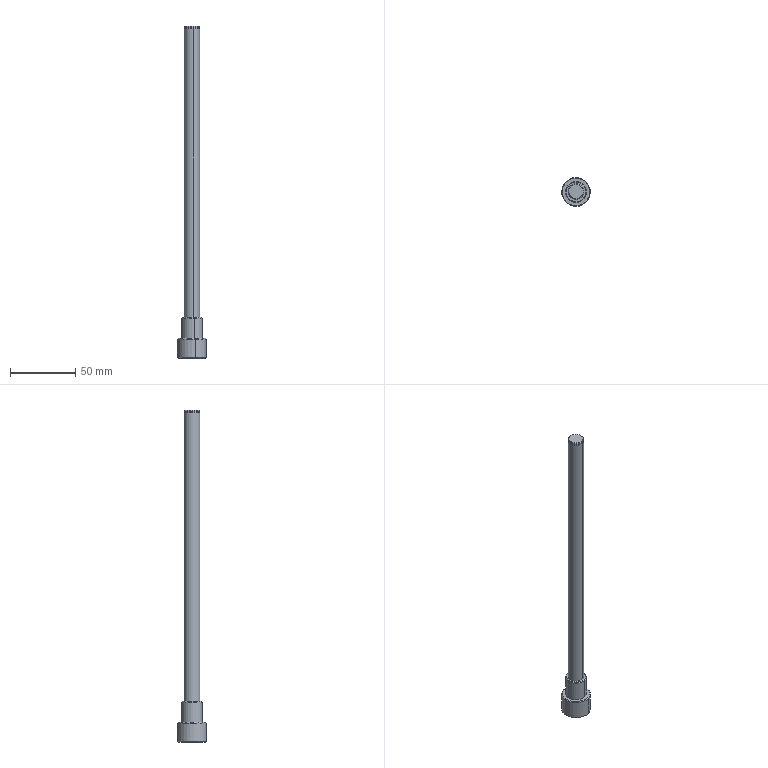Component | SolidWorks | JYTBJ-HeaderRollerBody-1_JYTBJ-HeaderRollerAxis-1 | 1 solid | 28 faces | box 22 x 22 x 254 mm | volume 33731 mm3 | cylinder 12 | cone 10 | plane 6 | commonest cylinder face diameters 12 x4 11 x2 5 x2 16 x2 22 x2
STEP:
#1=COLOUR_RGB('',0.7922,0.8196,0.9333);
#2=FILL_AREA_STYLE_COLOUR('',#1);
#3=FILL_AREA_STYLE('',(#2));
#4=SURFACE_STYLE_FILL_AREA(#3);
#5=SURFACE_SIDE_STYLE('',(#4));
#6=SURFACE_STYLE_USAGE(.BOTH.,#5);
#7=PRESENTATION_STYLE_ASSIGNMENT((#6));
#8=CARTESIAN_POINT('',(-7.808,6.896,10.63));
#9=VERTEX_POINT('',#8);
#10=CARTESIAN_POINT('',(-7.915,7.357,10.63));
#11=VERTEX_POINT('',#10);
#12=CARTESIAN_POINT('',(-7.862,7.126,10.63));
#13=DIRECTION('',(-0.,0.,-1.));
#14=DIRECTION('',(0.2266,-0.974,0.));
#15=AXIS2_PLACEMENT_3D('',#12,#13,#14);
#16=CIRCLE('',#15,0.2362);
#17=EDGE_CURVE('',#9,#11,#16,.T.);
#18=ORIENTED_EDGE('',*,*,#17,.T.);
#19=CARTESIAN_POINT('',(-7.915,7.357,1.929));
#20=VERTEX_POINT('',#19);
#21=CARTESIAN_POINT('',(-7.915,7.357,10.394));
#22=DIRECTION('',(-0.,0.,-1.));
#23=VECTOR('',#22,39.37);
#24=LINE('',#21,#23);
#25=EDGE_CURVE('',#11,#20,#24,.T.);
#26=ORIENTED_EDGE('',*,*,#25,.T.);
#27=CARTESIAN_POINT('',(-7.808,6.896,1.929));
#28=VERTEX_POINT('',#27);
#29=CARTESIAN_POINT('',(-7.862,7.126,1.929));
#30=DIRECTION('',(0.,-0.,1.));
#31=DIRECTION('',(-0.2266,0.974,0.));
#32=AXIS2_PLACEMENT_3D('',#29,#30,#31);
#33=CIRCLE('',#32,0.2362);
#34=EDGE_CURVE('',#20,#28,#33,.T.);
#35=ORIENTED_EDGE('',*,*,#34,.T.);
#36=CARTESIAN_POINT('',(-7.808,6.896,10.394));
#37=DIRECTION('',(-0.,0.,-1.));
#38=VECTOR('',#37,39.37);
#39=LINE('',#36,#38);
#40=EDGE_CURVE('',#9,#28,#39,.T.);
#41=ORIENTED_EDGE('',*,*,#40,.F.);
#42=EDGE_LOOP('',(#18,#26,#35,#41));
#43=FACE_OUTER_BOUND('',#42,.T.);
#44=CARTESIAN_POINT('',(-7.862,7.126,10.394));
#45=DIRECTION('',(-0.,0.,-1.));
#46=DIRECTION('',(0.2266,-0.974,0.));
#47=AXIS2_PLACEMENT_3D('',#44,#45,#46);
#48=CYLINDRICAL_SURFACE('',#47,0.2362);
#49=ADVANCED_FACE('',(#43),#48,.T.);
#50=CARTESIAN_POINT('',(-7.911,7.337,10.63));
#51=VERTEX_POINT('',#50);
#52=CARTESIAN_POINT('',(-7.813,6.916,10.63));
#53=VERTEX_POINT('',#52);
#54=CARTESIAN_POINT('',(-7.862,7.126,10.63));
#55=DIRECTION('',(0.,-0.,1.));
#56=DIRECTION('',(-0.2266,0.974,0.));
#57=AXIS2_PLACEMENT_3D('',#54,#55,#56);
#58=CIRCLE('',#57,0.2165);
#59=EDGE_CURVE('',#51,#53,#58,.T.);
#60=ORIENTED_EDGE('',*,*,#59,.T.);
#61=CARTESIAN_POINT('',(-7.813,6.916,10.669));
#62=VERTEX_POINT('',#61);
#63=CARTESIAN_POINT('',(-7.813,6.916,10.709));
#64=DIRECTION('',(0.,-0.,1.));
#65=VECTOR('',#64,39.37);
#66=LINE('',#63,#65);
#67=EDGE_CURVE('',#53,#62,#66,.T.);
#68=ORIENTED_EDGE('',*,*,#67,.T.);
#69=CARTESIAN_POINT('',(-7.911,7.337,10.669));
#70=VERTEX_POINT('',#69);
#71=CARTESIAN_POINT('',(-7.862,7.126,10.669));
#72=DIRECTION('',(0.,-0.,1.));
#73=DIRECTION('',(-0.2266,0.974,0.));
#74=AXIS2_PLACEMENT_3D('',#71,#72,#73);
#75=CIRCLE('',#74,0.2165);
#76=EDGE_CURVE('',#70,#62,#75,.T.);
#77=ORIENTED_EDGE('',*,*,#76,.F.);
#78=CARTESIAN_POINT('',(-7.911,7.337,10.709));
#79=DIRECTION('',(0.,-0.,1.));
#80=VECTOR('',#79,39.37);
#81=LINE('',#78,#80);
#82=EDGE_CURVE('',#51,#70,#81,.T.);
#83=ORIENTED_EDGE('',*,*,#82,.F.);
#84=EDGE_LOOP('',(#60,#68,#77,#83));
#85=FACE_OUTER_BOUND('',#84,.T.);
#86=CARTESIAN_POINT('',(-7.862,7.126,10.709));
#87=DIRECTION('',(0.,-0.,1.));
#88=DIRECTION('',(-0.2266,0.974,0.));
#89=AXIS2_PLACEMENT_3D('',#86,#87,#88);
#90=CYLINDRICAL_SURFACE('',#89,0.2165);
#91=ADVANCED_FACE('',(#85),#90,.T.);
#92=CARTESIAN_POINT('',(-7.808,6.896,10.689));
#93=VERTEX_POINT('',#92);
#94=CARTESIAN_POINT('',(-7.915,7.357,10.689));
#95=VERTEX_POINT('',#94);
#96=CARTESIAN_POINT('',(-7.862,7.126,10.689));
#97=DIRECTION('',(-0.,0.,-1.));
#98=DIRECTION('',(-0.2266,0.974,0.));
#99=AXIS2_PLACEMENT_3D('',#96,#97,#98);
#100=CIRCLE('',#99,0.2362);
#101=EDGE_CURVE('',#93,#95,#100,.T.);
#102=ORIENTED_EDGE('',*,*,#101,.T.);
#103=CARTESIAN_POINT('',(-7.915,7.357,10.669));
#104=VERTEX_POINT('',#103);
#105=CARTESIAN_POINT('',(-7.915,7.357,10.394));
#106=DIRECTION('',(-0.,0.,-1.));
#107=VECTOR('',#106,39.37);
#108=LINE('',#105,#107);
#109=EDGE_CURVE('',#95,#104,#108,.T.);
#110=ORIENTED_EDGE('',*,*,#109,.T.);
#111=CARTESIAN_POINT('',(-7.808,6.896,10.669));
#112=VERTEX_POINT('',#111);
#113=CARTESIAN_POINT('',(-7.862,7.126,10.669));
#114=DIRECTION('',(0.,-0.,1.));
#115=DIRECTION('',(-0.2266,0.974,0.));
#116=AXIS2_PLACEMENT_3D('',#113,#114,#115);
#117=CIRCLE('',#116,0.2362);
#118=EDGE_CURVE('',#104,#112,#117,.T.);
#119=ORIENTED_EDGE('',*,*,#118,.T.);
#120=CARTESIAN_POINT('',(-7.808,6.896,10.394));
#121=DIRECTION('',(-0.,0.,-1.));
#122=VECTOR('',#121,39.37);
#123=LINE('',#120,#122);
#124=EDGE_CURVE('',#93,#112,#123,.T.);
#125=ORIENTED_EDGE('',*,*,#124,.F.);
#126=EDGE_LOOP('',(#102,#110,#119,#125));
#127=FACE_OUTER_BOUND('',#126,.T.);
#128=CARTESIAN_POINT('',(-7.862,7.126,10.394));
#129=DIRECTION('',(-0.,0.,-1.));
#130=DIRECTION('',(0.2266,-0.974,0.));
#131=AXIS2_PLACEMENT_3D('',#128,#129,#130);
#132=CYLINDRICAL_SURFACE('',#131,0.2362);
#133=ADVANCED_FACE('',(#127),#132,.T.);
#134=CARTESIAN_POINT('',(-7.911,7.337,10.709));
#135=VERTEX_POINT('',#134);
#136=CARTESIAN_POINT('',(-7.813,6.916,10.709));
#137=VERTEX_POINT('',#136);
#138=CARTESIAN_POINT('',(-7.862,7.126,10.709));
#139=DIRECTION('',(0.,-0.,1.));
#140=DIRECTION('',(-0.2266,0.974,0.));
#141=AXIS2_PLACEMENT_3D('',#138,#139,#140);
#142=CIRCLE('',#141,0.2165);
#143=EDGE_CURVE('',#135,#137,#142,.T.);
#144=ORIENTED_EDGE('',*,*,#143,.F.);
#145=CARTESIAN_POINT('',(-7.911,7.337,10.709));
#146=DIRECTION('',(-0.1602,0.6887,-0.7071));
#147=VECTOR('',#146,39.37);
#148=LINE('',#145,#147);
#149=EDGE_CURVE('',#135,#95,#148,.T.);
#150=ORIENTED_EDGE('',*,*,#149,.T.);
#151=ORIENTED_EDGE('',*,*,#101,.F.);
#152=CARTESIAN_POINT('',(-7.813,6.916,10.709));
#153=DIRECTION('',(0.1602,-0.6887,-0.7071));
#154=VECTOR('',#153,39.37);
#155=LINE('',#152,#154);
#156=EDGE_CURVE('',#137,#93,#155,.T.);
#157=ORIENTED_EDGE('',*,*,#156,.F.);
#158=EDGE_LOOP('',(#144,#150,#151,#157));
#159=FACE_OUTER_BOUND('',#158,.T.);
#160=CARTESIAN_POINT('',(-7.862,7.126,10.709));
#161=DIRECTION('',(-0.,0.,-1.));
#162=DIRECTION('',(0.2266,-0.974,0.));
#163=AXIS2_PLACEMENT_3D('',#160,#161,#162);
#164=CONICAL_SURFACE('',#163,0.2165,0.7854);
#165=ADVANCED_FACE('',(#159),#164,.T.);
#166=CARTESIAN_POINT('',(-7.884,7.222,1.417));
#167=VERTEX_POINT('',#166);
#168=CARTESIAN_POINT('',(-7.84,7.031,1.417));
#169=VERTEX_POINT('',#168);
#170=CARTESIAN_POINT('',(-7.862,7.126,1.417));
#171=DIRECTION('',(-0.,0.,-1.));
#172=DIRECTION('',(0.2266,-0.974,0.));
#173=AXIS2_PLACEMENT_3D('',#170,#171,#172);
#174=CIRCLE('',#173,0.09843);
#175=EDGE_CURVE('',#167,#169,#174,.T.);
#176=ORIENTED_EDGE('',*,*,#175,.F.);
#177=CARTESIAN_POINT('',(-7.884,7.222,0.7087));
#178=VERTEX_POINT('',#177);
#179=CARTESIAN_POINT('',(-7.884,7.222,0.7087));
#180=DIRECTION('',(-0.,0.,-1.));
#181=VECTOR('',#180,39.37);
#182=LINE('',#179,#181);
#183=EDGE_CURVE('',#167,#178,#182,.T.);
#184=ORIENTED_EDGE('',*,*,#183,.T.);
#185=CARTESIAN_POINT('',(-7.84,7.031,0.7087));
#186=VERTEX_POINT('',#185);
#187=CARTESIAN_POINT('',(-7.862,7.126,0.7087));
#188=DIRECTION('',(-0.,0.,-1.));
#189=DIRECTION('',(0.2266,-0.974,0.));
#190=AXIS2_PLACEMENT_3D('',#187,#188,#189);
#191=CIRCLE('',#190,0.09843);
#192=EDGE_CURVE('',#178,#186,#191,.T.);
#193=ORIENTED_EDGE('',*,*,#192,.T.);
#194=CARTESIAN_POINT('',(-7.84,7.031,0.7087));
#195=DIRECTION('',(-0.,0.,-1.));
#196=VECTOR('',#195,39.37);
#197=LINE('',#194,#196);
#198=EDGE_CURVE('',#169,#186,#197,.T.);
#199=ORIENTED_EDGE('',*,*,#198,.F.);
#200=EDGE_LOOP('',(#176,#184,#193,#199));
#201=FACE_OUTER_BOUND('',#200,.T.);
#202=CARTESIAN_POINT('',(-7.862,7.126,0.7087));
#203=DIRECTION('',(-0.,0.,-1.));
#204=DIRECTION('',(0.2266,-0.974,0.));
#205=AXIS2_PLACEMENT_3D('',#202,#203,#204);
#206=CYLINDRICAL_SURFACE('',#205,0.09843);
#207=ADVANCED_FACE('',(#201),#206,.F.);
#208=CARTESIAN_POINT('',(-7.862,7.126,1.476));
#209=VERTEX_POINT('',#208);
#210=CARTESIAN_POINT('',(-7.84,7.031,1.417));
#211=DIRECTION('',(0.1943,-0.8349,-0.515));
#212=VECTOR('',#211,39.37);
#213=LINE('',#210,#212);
#214=EDGE_CURVE('',#209,#169,#213,.T.);
#215=ORIENTED_EDGE('',*,*,#214,.F.);
#216=CARTESIAN_POINT('',(-7.884,7.222,1.417));
#217=DIRECTION('',(-0.1943,0.8349,-0.515));
#218=VECTOR('',#217,39.37);
#219=LINE('',#216,#218);
#220=EDGE_CURVE('',#209,#167,#219,.T.);
#221=ORIENTED_EDGE('',*,*,#220,.T.);
#222=ORIENTED_EDGE('',*,*,#175,.T.);
#223=EDGE_LOOP('',(#215,#221,#222));
#224=FACE_OUTER_BOUND('',#223,.T.);
#225=CARTESIAN_POINT('',(-7.862,7.126,1.417));
#226=DIRECTION('',(-0.,0.,-1.));
#227=DIRECTION('',(0.2266,-0.974,0.));
#228=AXIS2_PLACEMENT_3D('',#225,#226,#227);
#229=CONICAL_SURFACE('',#228,0.09843,1.03);
#230=ADVANCED_FACE('',(#224),#229,.F.);
#231=CARTESIAN_POINT('',(-7.768,6.724,0.7087));
#232=VERTEX_POINT('',#231);
#233=CARTESIAN_POINT('',(-7.956,7.529,0.7087));
#234=VERTEX_POINT('',#233);
#235=CARTESIAN_POINT('',(-7.862,7.126,0.7087));
#236=DIRECTION('',(-0.,0.,-1.));
#237=DIRECTION('',(-0.2266,0.974,0.));
#238=AXIS2_PLACEMENT_3D('',#235,#236,#237);
#239=CIRCLE('',#238,0.4134);
#240=EDGE_CURVE('',#232,#234,#239,.T.);
#241=ORIENTED_EDGE('',*,*,#240,.F.);
#242=CARTESIAN_POINT('',(-7.764,6.705,0.7283));
#243=VERTEX_POINT('',#242);
#244=CARTESIAN_POINT('',(-7.764,6.705,0.7283));
#245=DIRECTION('',(0.1602,-0.6887,0.7071));
#246=VECTOR('',#245,39.37);
#247=LINE('',#244,#246);
#248=EDGE_CURVE('',#232,#243,#247,.T.);
#249=ORIENTED_EDGE('',*,*,#248,.T.);
#250=CARTESIAN_POINT('',(-7.96,7.548,0.7283));
#251=VERTEX_POINT('',#250);
#252=CARTESIAN_POINT('',(-7.862,7.126,0.7283));
#253=DIRECTION('',(0.,-0.,1.));
#254=DIRECTION('',(-0.2266,0.974,0.));
#255=AXIS2_PLACEMENT_3D('',#252,#253,#254);
#256=CIRCLE('',#255,0.4331);
#257=EDGE_CURVE('',#251,#243,#256,.T.);
#258=ORIENTED_EDGE('',*,*,#257,.F.);
#259=CARTESIAN_POINT('',(-7.96,7.548,0.7283));
#260=DIRECTION('',(-0.1602,0.6887,0.7071));
#261=VECTOR('',#260,39.37);
#262=LINE('',#259,#261);
#263=EDGE_CURVE('',#234,#251,#262,.T.);
#264=ORIENTED_EDGE('',*,*,#263,.F.);
#265=EDGE_LOOP('',(#241,#249,#258,#264));
#266=FACE_OUTER_BOUND('',#265,.T.);
#267=CARTESIAN_POINT('',(-7.862,7.126,0.7283));
#268=DIRECTION('',(0.,-0.,1.));
#269=DIRECTION('',(-0.2266,0.974,0.));
#270=AXIS2_PLACEMENT_3D('',#267,#268,#269);
#271=CONICAL_SURFACE('',#270,0.4331,0.7854);
#272=ADVANCED_FACE('',(#266),#271,.T.);
#273=CARTESIAN_POINT('',(-7.956,7.529,1.299));
#274=VERTEX_POINT('',#273);
#275=CARTESIAN_POINT('',(-7.768,6.724,1.299));
#276=VERTEX_POINT('',#275);
#277=CARTESIAN_POINT('',(-7.862,7.126,1.299));
#278=DIRECTION('',(0.,-0.,1.));
#279=DIRECTION('',(-0.2266,0.974,0.));
#280=AXIS2_PLACEMENT_3D('',#277,#278,#279);
#281=CIRCLE('',#280,0.4134);
#282=EDGE_CURVE('',#274,#276,#281,.T.);
#283=ORIENTED_EDGE('',*,*,#282,.F.);
#284=CARTESIAN_POINT('',(-7.96,7.548,1.28));
#285=VERTEX_POINT('',#284);
#286=CARTESIAN_POINT('',(-7.956,7.529,1.299));
#287=DIRECTION('',(-0.1602,0.6887,-0.7071));
#288=VECTOR('',#287,39.37);
#289=LINE('',#286,#288);
#290=EDGE_CURVE('',#274,#285,#289,.T.);
#291=ORIENTED_EDGE('',*,*,#290,.T.);
#292=CARTESIAN_POINT('',(-7.764,6.705,1.28));
#293=VERTEX_POINT('',#292);
#294=CARTESIAN_POINT('',(-7.862,7.126,1.28));
#295=DIRECTION('',(-0.,0.,-1.));
#296=DIRECTION('',(-0.2266,0.974,0.));
#297=AXIS2_PLACEMENT_3D('',#294,#295,#296);
#298=CIRCLE('',#297,0.4331);
#299=EDGE_CURVE('',#293,#285,#298,.T.);
#300=ORIENTED_EDGE('',*,*,#299,.F.);
#301=CARTESIAN_POINT('',(-7.768,6.724,1.299));
#302=DIRECTION('',(0.1602,-0.6887,-0.7071));
#303=VECTOR('',#302,39.37);
#304=LINE('',#301,#303);
#305=EDGE_CURVE('',#276,#293,#304,.T.);
#306=ORIENTED_EDGE('',*,*,#305,.F.);
#307=EDGE_LOOP('',(#283,#291,#300,#306));
#308=FACE_OUTER_BOUND('',#307,.T.);
#309=CARTESIAN_POINT('',(-7.862,7.126,1.299));
#310=DIRECTION('',(-0.,0.,-1.));
#311=DIRECTION('',(0.2266,-0.974,0.));
#312=AXIS2_PLACEMENT_3D('',#309,#310,#311);
#313=CONICAL_SURFACE('',#312,0.4134,0.7854);
#314=ADVANCED_FACE('',(#308),#313,.T.);
#315=CARTESIAN_POINT('',(-7.929,7.414,1.929));
#316=VERTEX_POINT('',#315);
#317=CARTESIAN_POINT('',(-7.795,6.839,1.929));
#318=VERTEX_POINT('',#317);
#319=CARTESIAN_POINT('',(-7.862,7.126,1.929));
#320=DIRECTION('',(0.,-0.,1.));
#321=DIRECTION('',(-0.2266,0.974,0.));
#322=AXIS2_PLACEMENT_3D('',#319,#320,#321);
#323=CIRCLE('',#322,0.2953);
#324=EDGE_CURVE('',#316,#318,#323,.T.);
#325=ORIENTED_EDGE('',*,*,#324,.F.);
#326=CARTESIAN_POINT('',(-7.933,7.433,1.909));
#327=VERTEX_POINT('',#326);
#328=CARTESIAN_POINT('',(-7.929,7.414,1.929));
#329=DIRECTION('',(-0.1602,0.6887,-0.7071));
#330=VECTOR('',#329,39.37);
#331=LINE('',#328,#330);
#332=EDGE_CURVE('',#316,#327,#331,.T.);
#333=ORIENTED_EDGE('',*,*,#332,.T.);
#334=CARTESIAN_POINT('',(-7.791,6.82,1.909));
#335=VERTEX_POINT('',#334);
#336=CARTESIAN_POINT('',(-7.862,7.126,1.909));
#337=DIRECTION('',(-0.,0.,-1.));
#338=DIRECTION('',(-0.2266,0.974,0.));
#339=AXIS2_PLACEMENT_3D('',#336,#337,#338);
#340=CIRCLE('',#339,0.315);
#341=EDGE_CURVE('',#335,#327,#340,.T.);
#342=ORIENTED_EDGE('',*,*,#341,.F.);
#343=CARTESIAN_POINT('',(-7.795,6.839,1.929));
#344=DIRECTION('',(0.1602,-0.6887,-0.7071));
#345=VECTOR('',#344,39.37);
#346=LINE('',#343,#345);
#347=EDGE_CURVE('',#318,#335,#346,.T.);
#348=ORIENTED_EDGE('',*,*,#347,.F.);
#349=EDGE_LOOP('',(#325,#333,#342,#348));
#350=FACE_OUTER_BOUND('',#349,.T.);
#351=CARTESIAN_POINT('',(-7.862,7.126,1.929));
#352=DIRECTION('',(-0.,0.,-1.));
#353=DIRECTION('',(0.2266,-0.974,0.));
#354=AXIS2_PLACEMENT_3D('',#351,#352,#353);
#355=CONICAL_SURFACE('',#354,0.2953,0.7854);
#356=ADVANCED_FACE('',(#350),#355,.T.);
#357=ORIENTED_EDGE('',*,*,#341,.T.);
#358=CARTESIAN_POINT('',(-7.933,7.433,1.299));
#359=VERTEX_POINT('',#358);
#360=CARTESIAN_POINT('',(-7.933,7.433,1.929));
#361=DIRECTION('',(-0.,0.,-1.));
#362=VECTOR('',#361,39.37);
#363=LINE('',#360,#362);
#364=EDGE_CURVE('',#327,#359,#363,.T.);
#365=ORIENTED_EDGE('',*,*,#364,.T.);
#366=CARTESIAN_POINT('',(-7.791,6.82,1.299));
#367=VERTEX_POINT('',#366);
#368=CARTESIAN_POINT('',(-7.862,7.126,1.299));
#369=DIRECTION('',(0.,-0.,1.));
#370=DIRECTION('',(-0.2266,0.974,0.));
#371=AXIS2_PLACEMENT_3D('',#368,#369,#370);
#372=CIRCLE('',#371,0.315);
#373=EDGE_CURVE('',#359,#367,#372,.T.);
#374=ORIENTED_EDGE('',*,*,#373,.T.);
#375=CARTESIAN_POINT('',(-7.791,6.82,1.929));
#376=DIRECTION('',(-0.,0.,-1.));
#377=VECTOR('',#376,39.37);
#378=LINE('',#375,#377);
#379=EDGE_CURVE('',#335,#367,#378,.T.);
#380=ORIENTED_EDGE('',*,*,#379,.F.);
#381=EDGE_LOOP('',(#357,#365,#374,#380));
#382=FACE_OUTER_BOUND('',#381,.T.);
#383=CARTESIAN_POINT('',(-7.862,7.126,1.929));
#384=DIRECTION('',(-0.,0.,-1.));
#385=DIRECTION('',(0.2266,-0.974,0.));
#386=AXIS2_PLACEMENT_3D('',#383,#384,#385);
#387=CYLINDRICAL_SURFACE('',#386,0.315);
#388=ADVANCED_FACE('',(#382),#387,.T.);
#389=ORIENTED_EDGE('',*,*,#299,.T.);
#390=CARTESIAN_POINT('',(-7.96,7.548,1.299));
#391=DIRECTION('',(-0.,0.,-1.));
#392=VECTOR('',#391,39.37);
#393=LINE('',#390,#392);
#394=EDGE_CURVE('',#285,#251,#393,.T.);
#395=ORIENTED_EDGE('',*,*,#394,.T.);
#396=ORIENTED_EDGE('',*,*,#257,.T.);
#397=CARTESIAN_POINT('',(-7.764,6.705,1.299));
#398=DIRECTION('',(-0.,0.,-1.));
#399=VECTOR('',#398,39.37);
#400=LINE('',#397,#399);
#401=EDGE_CURVE('',#293,#243,#400,.T.);
#402=ORIENTED_EDGE('',*,*,#401,.F.);
#403=EDGE_LOOP('',(#389,#395,#396,#402));
#404=FACE_OUTER_BOUND('',#403,.T.);
#405=CARTESIAN_POINT('',(-7.862,7.126,1.299));
#406=DIRECTION('',(-0.,0.,-1.));
#407=DIRECTION('',(0.2266,-0.974,0.));
#408=AXIS2_PLACEMENT_3D('',#405,#406,#407);
#409=CYLINDRICAL_SURFACE('',#408,0.4331);
#410=ADVANCED_FACE('',(#404),#409,.T.);
#411=CARTESIAN_POINT('',(-7.862,7.126,1.299));
#412=DIRECTION('',(0.,-0.,1.));
#413=DIRECTION('',(-0.2266,0.974,0.));
#414=AXIS2_PLACEMENT_3D('',#411,#412,#413);
#415=CIRCLE('',#414,0.4134);
#416=EDGE_CURVE('',#276,#274,#415,.T.);
#417=ORIENTED_EDGE('',*,*,#416,.T.);
#418=ORIENTED_EDGE('',*,*,#282,.T.);
#419=EDGE_LOOP('',(#417,#418));
#420=FACE_OUTER_BOUND('',#419,.T.);
#421=CARTESIAN_POINT('',(-7.862,7.126,1.299));
#422=DIRECTION('',(0.,-0.,1.));
#423=DIRECTION('',(-0.2266,0.974,0.));
#424=AXIS2_PLACEMENT_3D('',#421,#422,#423);
#425=CIRCLE('',#424,0.315);
#426=EDGE_CURVE('',#367,#359,#425,.T.);
#427=ORIENTED_EDGE('',*,*,#426,.F.);
#428=ORIENTED_EDGE('',*,*,#373,.F.);
#429=EDGE_LOOP('',(#427,#428));
#430=FACE_BOUND('',#429,.T.);
#431=CARTESIAN_POINT('',(-7.862,7.126,1.299));
#432=DIRECTION('',(0.,-0.,1.));
#433=DIRECTION('',(-0.2266,0.974,0.));
#434=AXIS2_PLACEMENT_3D('',#431,#432,#433);
#435=PLANE('',#434);
#436=ADVANCED_FACE('',(#420,#430),#435,.T.);
#437=ORIENTED_EDGE('',*,*,#394,.F.);
#438=CARTESIAN_POINT('',(-7.862,7.126,1.28));
#439=DIRECTION('',(-0.,0.,-1.));
#440=DIRECTION('',(-0.2266,0.974,0.));
#441=AXIS2_PLACEMENT_3D('',#438,#439,#440);
#442=CIRCLE('',#441,0.4331);
#443=EDGE_CURVE('',#285,#293,#442,.T.);
#444=ORIENTED_EDGE('',*,*,#443,.T.);
#445=ORIENTED_EDGE('',*,*,#401,.T.);
#446=CARTESIAN_POINT('',(-7.862,7.126,0.7283));
#447=DIRECTION('',(0.,-0.,1.));
#448=DIRECTION('',(-0.2266,0.974,0.));
#449=AXIS2_PLACEMENT_3D('',#446,#447,#448);
#450=CIRCLE('',#449,0.4331);
#451=EDGE_CURVE('',#243,#251,#450,.T.);
#452=ORIENTED_EDGE('',*,*,#451,.T.);
#453=EDGE_LOOP('',(#437,#444,#445,#452));
#454=FACE_OUTER_BOUND('',#453,.T.);
#455=CARTESIAN_POINT('',(-7.862,7.126,1.299));
#456=DIRECTION('',(-0.,0.,-1.));
#457=DIRECTION('',(0.2266,-0.974,0.));
#458=AXIS2_PLACEMENT_3D('',#455,#456,#457);
#459=CYLINDRICAL_SURFACE('',#458,0.4331);
#460=ADVANCED_FACE('',(#454),#459,.T.);
#461=CARTESIAN_POINT('',(-7.862,7.126,0.7087));
#462=DIRECTION('',(-0.,0.,-1.));
#463=DIRECTION('',(0.2266,-0.974,0.));
#464=AXIS2_PLACEMENT_3D('',#461,#462,#463);
#465=CIRCLE('',#464,0.09843);
#466=EDGE_CURVE('',#186,#178,#465,.T.);
#467=ORIENTED_EDGE('',*,*,#466,.F.);
#468=ORIENTED_EDGE('',*,*,#192,.F.);
#469=EDGE_LOOP('',(#467,#468));
#470=FACE_BOUND('',#469,.T.);
#471=CARTESIAN_POINT('',(-7.862,7.126,0.7087));
#472=DIRECTION('',(-0.,0.,-1.));
#473=DIRECTION('',(-0.2266,0.974,0.));
#474=AXIS2_PLACEMENT_3D('',#471,#472,#473);
#475=CIRCLE('',#474,0.4134);
#476=EDGE_CURVE('',#234,#232,#475,.T.);
#477=ORIENTED_EDGE('',*,*,#476,.T.);
#478=ORIENTED_EDGE('',*,*,#240,.T.);
#479=EDGE_LOOP('',(#477,#478));
#480=FACE_OUTER_BOUND('',#479,.T.);
#481=CARTESIAN_POINT('',(-7.862,7.126,0.7087));
#482=DIRECTION('',(0.,-0.,1.));
#483=DIRECTION('',(-0.2266,0.974,0.));
#484=AXIS2_PLACEMENT_3D('',#481,#482,#483);
#485=PLANE('',#484);
#486=ADVANCED_FACE('',(#470,#480),#485,.F.);
#487=ORIENTED_EDGE('',*,*,#364,.F.);
#488=CARTESIAN_POINT('',(-7.862,7.126,1.909));
#489=DIRECTION('',(-0.,0.,-1.));
#490=DIRECTION('',(-0.2266,0.974,0.));
#491=AXIS2_PLACEMENT_3D('',#488,#489,#490);
#492=CIRCLE('',#491,0.315);
#493=EDGE_CURVE('',#327,#335,#492,.T.);
#494=ORIENTED_EDGE('',*,*,#493,.T.);
#495=ORIENTED_EDGE('',*,*,#379,.T.);
#496=ORIENTED_EDGE('',*,*,#426,.T.);
#497=EDGE_LOOP('',(#487,#494,#495,#496));
#498=FACE_OUTER_BOUND('',#497,.T.);
#499=CARTESIAN_POINT('',(-7.862,7.126,1.929));
#500=DIRECTION('',(-0.,0.,-1.));
#501=DIRECTION('',(0.2266,-0.974,0.));
#502=AXIS2_PLACEMENT_3D('',#499,#500,#501);
#503=CYLINDRICAL_SURFACE('',#502,0.315);
#504=ADVANCED_FACE('',(#498),#503,.T.);
#505=ORIENTED_EDGE('',*,*,#332,.F.);
#506=CARTESIAN_POINT('',(-7.862,7.126,1.929));
#507=DIRECTION('',(0.,-0.,1.));
#508=DIRECTION('',(-0.2266,0.974,0.));
#509=AXIS2_PLACEMENT_3D('',#506,#507,#508);
#510=CIRCLE('',#509,0.2953);
#511=EDGE_CURVE('',#318,#316,#510,.T.);
#512=ORIENTED_EDGE('',*,*,#511,.F.);
#513=ORIENTED_EDGE('',*,*,#347,.T.);
#514=ORIENTED_EDGE('',*,*,#493,.F.);
#515=EDGE_LOOP('',(#505,#512,#513,#514));
#516=FACE_OUTER_BOUND('',#515,.T.);
#517=CARTESIAN_POINT('',(-7.862,7.126,1.929));
#518=DIRECTION('',(-0.,0.,-1.));
#519=DIRECTION('',(0.2266,-0.974,0.));
#520=AXIS2_PLACEMENT_3D('',#517,#518,#519);
#521=CONICAL_SURFACE('',#520,0.2953,0.7854);
#522=ADVANCED_FACE('',(#516),#521,.T.);
#523=ORIENTED_EDGE('',*,*,#290,.F.);
#524=ORIENTED_EDGE('',*,*,#416,.F.);
#525=ORIENTED_EDGE('',*,*,#305,.T.);
#526=ORIENTED_EDGE('',*,*,#443,.F.);
#527=EDGE_LOOP('',(#523,#524,#525,#526));
#528=FACE_OUTER_BOUND('',#527,.T.);
#529=CARTESIAN_POINT('',(-7.862,7.126,1.299));
#530=DIRECTION('',(-0.,0.,-1.));
#531=DIRECTION('',(0.2266,-0.974,0.));
#532=AXIS2_PLACEMENT_3D('',#529,#530,#531);
#533=CONICAL_SURFACE('',#532,0.4134,0.7854);
#534=ADVANCED_FACE('',(#528),#533,.T.);
#535=ORIENTED_EDGE('',*,*,#248,.F.);
#536=ORIENTED_EDGE('',*,*,#476,.F.);
#537=ORIENTED_EDGE('',*,*,#263,.T.);
#538=ORIENTED_EDGE('',*,*,#451,.F.);
#539=EDGE_LOOP('',(#535,#536,#537,#538));
#540=FACE_OUTER_BOUND('',#539,.T.);
#541=CARTESIAN_POINT('',(-7.862,7.126,0.7283));
#542=DIRECTION('',(0.,-0.,1.));
#543=DIRECTION('',(-0.2266,0.974,0.));
#544=AXIS2_PLACEMENT_3D('',#541,#542,#543);
#545=CONICAL_SURFACE('',#544,0.4331,0.7854);
#546=ADVANCED_FACE('',(#540),#545,.T.);
#547=ORIENTED_EDGE('',*,*,#220,.F.);
#548=ORIENTED_EDGE('',*,*,#214,.T.);
#549=CARTESIAN_POINT('',(-7.862,7.126,1.417));
#550=DIRECTION('',(-0.,0.,-1.));
#551=DIRECTION('',(0.2266,-0.974,0.));
#552=AXIS2_PLACEMENT_3D('',#549,#550,#551);
#553=CIRCLE('',#552,0.09843);
#554=EDGE_CURVE('',#169,#167,#553,.T.);
#555=ORIENTED_EDGE('',*,*,#554,.T.);
#556=EDGE_LOOP('',(#547,#548,#555));
#557=FACE_OUTER_BOUND('',#556,.T.);
#558=CARTESIAN_POINT('',(-7.862,7.126,1.417));
#559=DIRECTION('',(-0.,0.,-1.));
#560=DIRECTION('',(0.2266,-0.974,0.));
#561=AXIS2_PLACEMENT_3D('',#558,#559,#560);
#562=CONICAL_SURFACE('',#561,0.09843,1.03);
#563=ADVANCED_FACE('',(#557),#562,.F.);
#564=ORIENTED_EDGE('',*,*,#183,.F.);
#565=ORIENTED_EDGE('',*,*,#554,.F.);
#566=ORIENTED_EDGE('',*,*,#198,.T.);
#567=ORIENTED_EDGE('',*,*,#466,.T.);
#568=EDGE_LOOP('',(#564,#565,#566,#567));
#569=FACE_OUTER_BOUND('',#568,.T.);
#570=CARTESIAN_POINT('',(-7.862,7.126,0.7087));
#571=DIRECTION('',(-0.,0.,-1.));
#572=DIRECTION('',(0.2266,-0.974,0.));
#573=AXIS2_PLACEMENT_3D('',#570,#571,#572);
#574=CYLINDRICAL_SURFACE('',#573,0.09843);
#575=ADVANCED_FACE('',(#569),#574,.F.);
#576=CARTESIAN_POINT('',(-7.862,7.126,1.929));
#577=DIRECTION('',(0.,-0.,1.));
#578=DIRECTION('',(-0.2266,0.974,0.));
#579=AXIS2_PLACEMENT_3D('',#576,#577,#578);
#580=CIRCLE('',#579,0.2362);
#581=EDGE_CURVE('',#28,#20,#580,.T.);
#582=ORIENTED_EDGE('',*,*,#581,.F.);
#583=ORIENTED_EDGE('',*,*,#34,.F.);
#584=EDGE_LOOP('',(#582,#583));
#585=FACE_BOUND('',#584,.T.);
#586=ORIENTED_EDGE('',*,*,#511,.T.);
#587=ORIENTED_EDGE('',*,*,#324,.T.);
#588=EDGE_LOOP('',(#586,#587));
#589=FACE_OUTER_BOUND('',#588,.T.);
#590=CARTESIAN_POINT('',(-7.862,7.126,1.929));
#591=DIRECTION('',(0.,-0.,1.));
#592=DIRECTION('',(-0.2266,0.974,0.));
#593=AXIS2_PLACEMENT_3D('',#590,#591,#592);
#594=PLANE('',#593);
#595=ADVANCED_FACE('',(#585,#589),#594,.T.);
#596=CARTESIAN_POINT('',(-7.862,7.126,10.709));
#597=DIRECTION('',(0.,-0.,1.));
#598=DIRECTION('',(-0.2266,0.974,0.));
#599=AXIS2_PLACEMENT_3D('',#596,#597,#598);
#600=CIRCLE('',#599,0.2165);
#601=EDGE_CURVE('',#137,#135,#600,.T.);
#602=ORIENTED_EDGE('',*,*,#601,.T.);
#603=ORIENTED_EDGE('',*,*,#143,.T.);
#604=EDGE_LOOP('',(#602,#603));
#605=FACE_OUTER_BOUND('',#604,.T.);
#606=CARTESIAN_POINT('',(-7.862,7.126,10.709));
#607=DIRECTION('',(0.,-0.,1.));
#608=DIRECTION('',(-0.2266,0.974,0.));
#609=AXIS2_PLACEMENT_3D('',#606,#607,#608);
#610=PLANE('',#609);
#611=ADVANCED_FACE('',(#605),#610,.T.);
#612=ORIENTED_EDGE('',*,*,#149,.F.);
#613=ORIENTED_EDGE('',*,*,#601,.F.);
#614=ORIENTED_EDGE('',*,*,#156,.T.);
#615=CARTESIAN_POINT('',(-7.862,7.126,10.689));
#616=DIRECTION('',(-0.,0.,-1.));
#617=DIRECTION('',(-0.2266,0.974,0.));
#618=AXIS2_PLACEMENT_3D('',#615,#616,#617);
#619=CIRCLE('',#618,0.2362);
#620=EDGE_CURVE('',#95,#93,#619,.T.);
#621=ORIENTED_EDGE('',*,*,#620,.F.);
#622=EDGE_LOOP('',(#612,#613,#614,#621));
#623=FACE_OUTER_BOUND('',#622,.T.);
#624=CARTESIAN_POINT('',(-7.862,7.126,10.709));
#625=DIRECTION('',(-0.,0.,-1.));
#626=DIRECTION('',(0.2266,-0.974,0.));
#627=AXIS2_PLACEMENT_3D('',#624,#625,#626);
#628=CONICAL_SURFACE('',#627,0.2165,0.7854);
#629=ADVANCED_FACE('',(#623),#628,.T.);
#630=ORIENTED_EDGE('',*,*,#109,.F.);
#631=ORIENTED_EDGE('',*,*,#620,.T.);
#632=ORIENTED_EDGE('',*,*,#124,.T.);
#633=CARTESIAN_POINT('',(-7.862,7.126,10.669));
#634=DIRECTION('',(0.,-0.,1.));
#635=DIRECTION('',(-0.2266,0.974,0.));
#636=AXIS2_PLACEMENT_3D('',#633,#634,#635);
#637=CIRCLE('',#636,0.2362);
#638=EDGE_CURVE('',#112,#104,#637,.T.);
#639=ORIENTED_EDGE('',*,*,#638,.T.);
#640=EDGE_LOOP('',(#630,#631,#632,#639));
#641=FACE_OUTER_BOUND('',#640,.T.);
#642=CARTESIAN_POINT('',(-7.862,7.126,10.394));
#643=DIRECTION('',(-0.,0.,-1.));
#644=DIRECTION('',(0.2266,-0.974,0.));
#645=AXIS2_PLACEMENT_3D('',#642,#643,#644);
#646=CYLINDRICAL_SURFACE('',#645,0.2362);
#647=ADVANCED_FACE('',(#641),#646,.T.);
#648=ORIENTED_EDGE('',*,*,#76,.T.);
#649=CARTESIAN_POINT('',(-7.862,7.126,10.669));
#650=DIRECTION('',(0.,-0.,1.));
#651=DIRECTION('',(-0.2266,0.974,0.));
#652=AXIS2_PLACEMENT_3D('',#649,#650,#651);
#653=CIRCLE('',#652,0.2165);
#654=EDGE_CURVE('',#62,#70,#653,.T.);
#655=ORIENTED_EDGE('',*,*,#654,.T.);
#656=EDGE_LOOP('',(#648,#655));
#657=FACE_BOUND('',#656,.T.);
#658=ORIENTED_EDGE('',*,*,#638,.F.);
#659=ORIENTED_EDGE('',*,*,#118,.F.);
#660=EDGE_LOOP('',(#658,#659));
#661=FACE_OUTER_BOUND('',#660,.T.);
#662=CARTESIAN_POINT('',(-8.096,7.072,10.669));
#663=DIRECTION('',(0.,-0.,1.));
#664=DIRECTION('',(-0.2266,0.974,0.));
#665=AXIS2_PLACEMENT_3D('',#662,#663,#664);
#666=PLANE('',#665);
#667=ADVANCED_FACE('',(#657,#661),#666,.F.);
#668=ORIENTED_EDGE('',*,*,#67,.F.);
#669=CARTESIAN_POINT('',(-7.862,7.126,10.63));
#670=DIRECTION('',(0.,-0.,1.));
#671=DIRECTION('',(-0.2266,0.974,0.));
#672=AXIS2_PLACEMENT_3D('',#669,#670,#671);
#673=CIRCLE('',#672,0.2165);
#674=EDGE_CURVE('',#53,#51,#673,.T.);
#675=ORIENTED_EDGE('',*,*,#674,.T.);
#676=ORIENTED_EDGE('',*,*,#82,.T.);
#677=ORIENTED_EDGE('',*,*,#654,.F.);
#678=EDGE_LOOP('',(#668,#675,#676,#677));
#679=FACE_OUTER_BOUND('',#678,.T.);
#680=CARTESIAN_POINT('',(-7.862,7.126,10.709));
#681=DIRECTION('',(0.,-0.,1.));
#682=DIRECTION('',(-0.2266,0.974,0.));
#683=AXIS2_PLACEMENT_3D('',#680,#681,#682);
#684=CYLINDRICAL_SURFACE('',#683,0.2165);
#685=ADVANCED_FACE('',(#679),#684,.T.);
#686=ORIENTED_EDGE('',*,*,#59,.F.);
#687=ORIENTED_EDGE('',*,*,#674,.F.);
#688=EDGE_LOOP('',(#686,#687));
#689=FACE_BOUND('',#688,.T.);
#690=ORIENTED_EDGE('',*,*,#17,.F.);
#691=CARTESIAN_POINT('',(-7.862,7.126,10.63));
#692=DIRECTION('',(-0.,0.,-1.));
#693=DIRECTION('',(0.2266,-0.974,0.));
#694=AXIS2_PLACEMENT_3D('',#691,#692,#693);
#695=CIRCLE('',#694,0.2362);
#696=EDGE_CURVE('',#11,#9,#695,.T.);
#697=ORIENTED_EDGE('',*,*,#696,.F.);
#698=EDGE_LOOP('',(#690,#697));
#699=FACE_OUTER_BOUND('',#698,.T.);
#700=CARTESIAN_POINT('',(-8.096,7.072,10.63));
#701=DIRECTION('',(-0.,0.,-1.));
#702=DIRECTION('',(0.2266,-0.974,-0.));
#703=AXIS2_PLACEMENT_3D('',#700,#701,#702);
#704=PLANE('',#703);
#705=ADVANCED_FACE('',(#689,#699),#704,.F.);
#706=ORIENTED_EDGE('',*,*,#25,.F.);
#707=ORIENTED_EDGE('',*,*,#696,.T.);
#708=ORIENTED_EDGE('',*,*,#40,.T.);
#709=ORIENTED_EDGE('',*,*,#581,.T.);
#710=EDGE_LOOP('',(#706,#707,#708,#709));
#711=FACE_OUTER_BOUND('',#710,.T.);
#712=CARTESIAN_POINT('',(-7.862,7.126,10.394));
#713=DIRECTION('',(-0.,0.,-1.));
#714=DIRECTION('',(0.2266,-0.974,0.));
#715=AXIS2_PLACEMENT_3D('',#712,#713,#714);
#716=CYLINDRICAL_SURFACE('',#715,0.2362);
#717=ADVANCED_FACE('',(#711),#716,.T.);
#718=CLOSED_SHELL('',(#49,#91,#133,#165,#207,#230,#272,#314,#356,#388,#410,#436,#460,#486,#504,#522,#534,#546,#563,#575,#595,#611,#629,#647,#667,#685,#705,#717));
#719=MANIFOLD_SOLID_BREP('',#718);
#720=STYLED_ITEM('',(#7),#719);
#721=PRESENTATION_LAYER_ASSIGNMENT('','',(#720));
#722=CARTESIAN_POINT('',(0.,0.,0.));
#723=DIRECTION('',(0.,0.,1.));
#724=DIRECTION('',(1.,0.,0.));
#725=AXIS2_PLACEMENT_3D('',#722,#723,#724);
#726=(LENGTH_UNIT()NAMED_UNIT(*)SI_UNIT($,.METRE.));
#727=LENGTH_MEASURE_WITH_UNIT(LENGTH_MEASURE(0.0254),#726);
#728=DIMENSIONAL_EXPONENTS(1.,0.,0.,0.,0.,0.,0.);
#729=(CONVERSION_BASED_UNIT('',#727)LENGTH_UNIT()NAMED_UNIT(#728));
#730=UNCERTAINTY_MEASURE_WITH_UNIT(LENGTH_MEASURE(0.00001),#729,'','');
#731=(NAMED_UNIT(*)PLANE_ANGLE_UNIT()SI_UNIT($,.RADIAN.));
#732=(NAMED_UNIT(*)SI_UNIT($,.STERADIAN.)SOLID_ANGLE_UNIT());
#733=(GEOMETRIC_REPRESENTATION_CONTEXT(3)GLOBAL_UNCERTAINTY_ASSIGNED_CONTEXT((#730))GLOBAL_UNIT_ASSIGNED_CONTEXT((#729,#731,#732))REPRESENTATION_CONTEXT('',''));
#734=ADVANCED_BREP_SHAPE_REPRESENTATION('',(#719,#725),#733);
#735=(LENGTH_UNIT()NAMED_UNIT(*)SI_UNIT($,.METRE.));
#736=LENGTH_MEASURE_WITH_UNIT(LENGTH_MEASURE(0.0254),#735);
#737=DIMENSIONAL_EXPONENTS(1.,0.,0.,0.,0.,0.,0.);
#738=(CONVERSION_BASED_UNIT('',#736)LENGTH_UNIT()NAMED_UNIT(#737));
#739=UNCERTAINTY_MEASURE_WITH_UNIT(LENGTH_MEASURE(0.00001),#738,'','');
#740=(NAMED_UNIT(*)PLANE_ANGLE_UNIT()SI_UNIT($,.RADIAN.));
#741=(NAMED_UNIT(*)SI_UNIT($,.STERADIAN.)SOLID_ANGLE_UNIT());
#742=(GEOMETRIC_REPRESENTATION_CONTEXT(3)GLOBAL_UNCERTAINTY_ASSIGNED_CONTEXT((#739))GLOBAL_UNIT_ASSIGNED_CONTEXT((#738,#740,#741))REPRESENTATION_CONTEXT('',''));
#743=MECHANICAL_DESIGN_GEOMETRIC_PRESENTATION_REPRESENTATION('',(#720),#742);